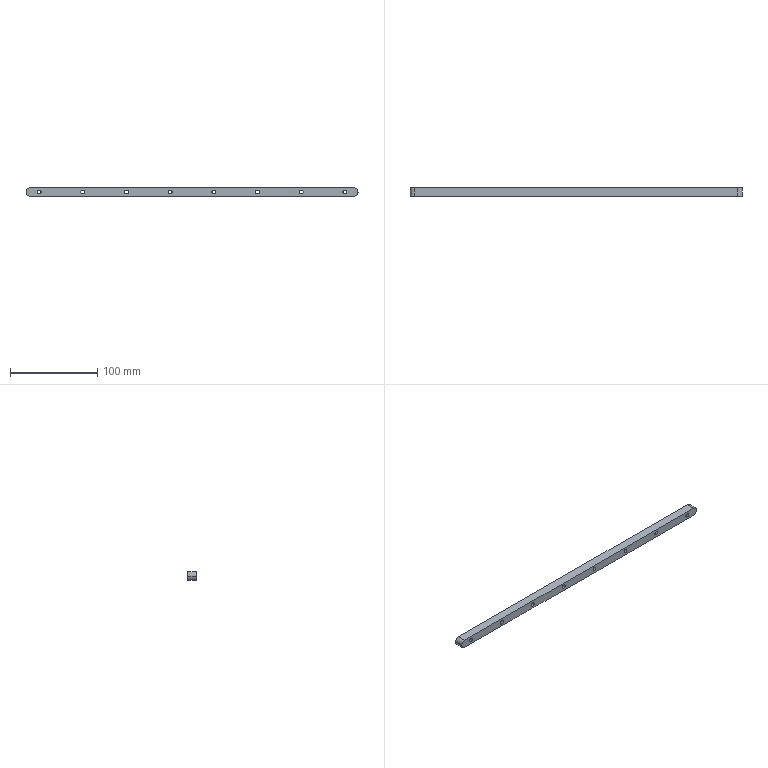Component | SolidWorks | 002MaterialPickingModuleA-1_004SidePlugModule-1_J-013-2 | 1 solid | 48 faces | volume 35304 mm3 | cylinder 36 | plane 12 | commonest cylinder face diameters 8 x16 4.5 x16 10 x4 | material 45